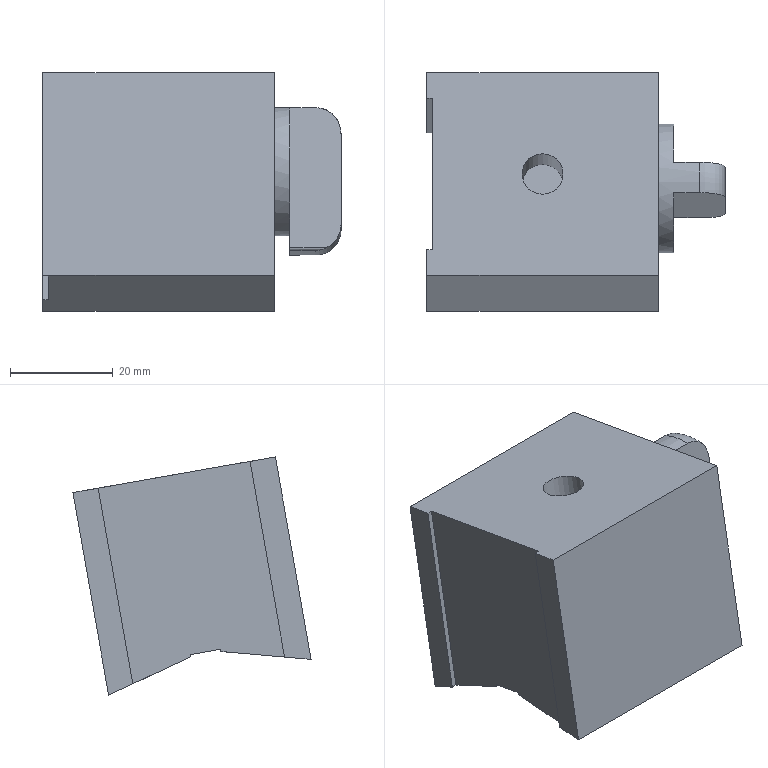Component | NX | MAGNETIC_BASE | 1 solid | 28 faces | volume 68573 mm3 | plane 22 | cylinder 5 | torus 1 | commonest cylinder face diameters 1 x2 25 x1 8 x1 10 x1